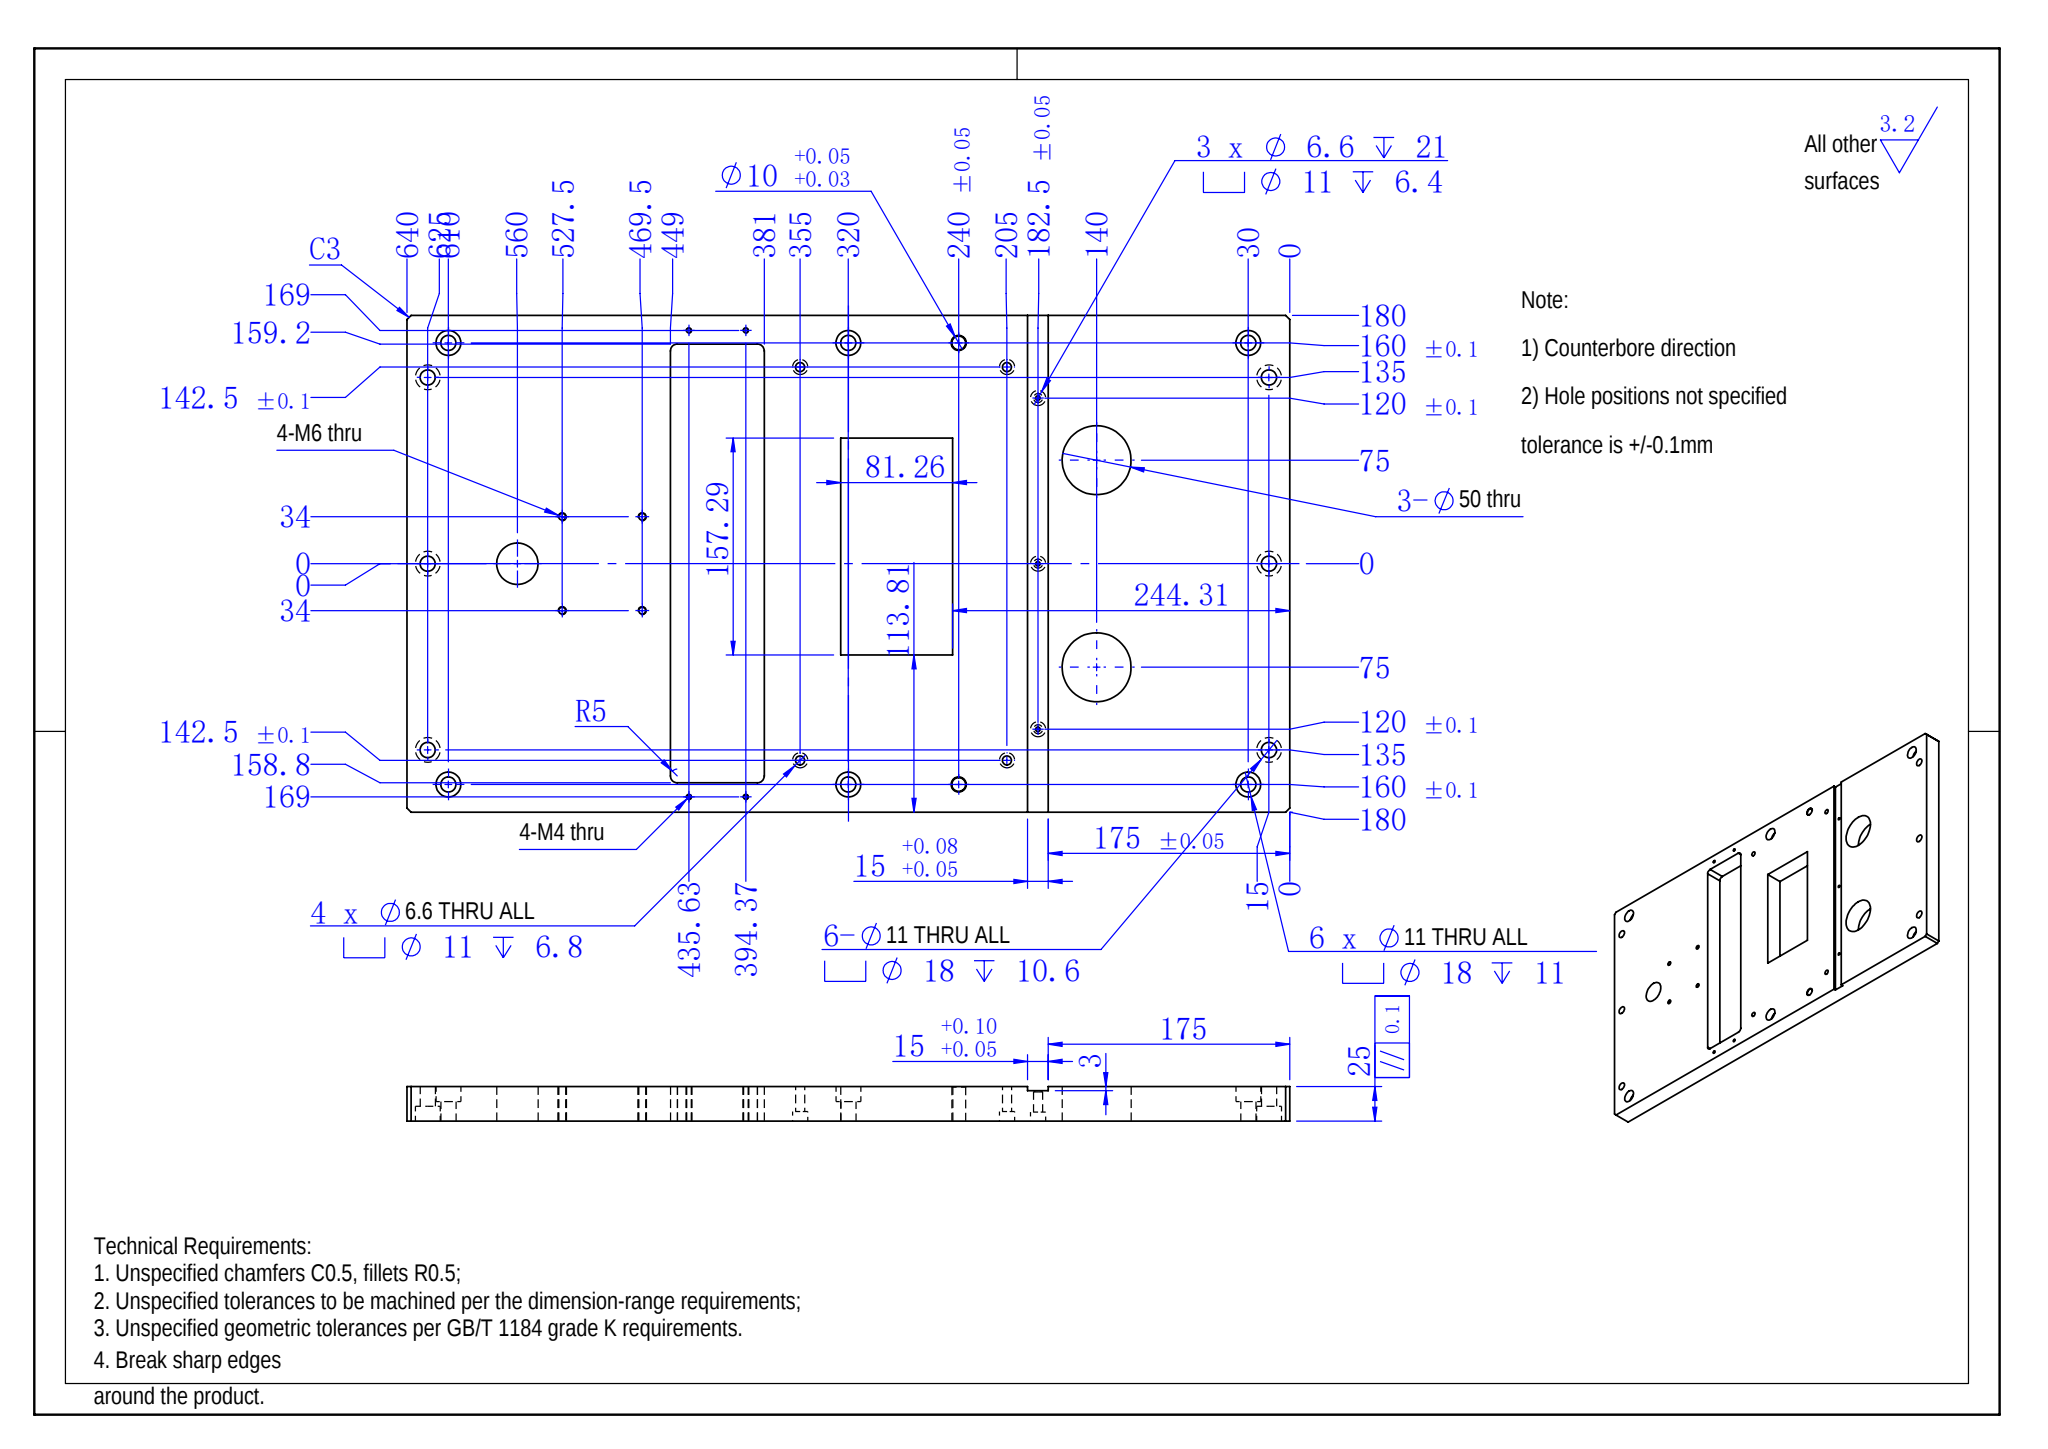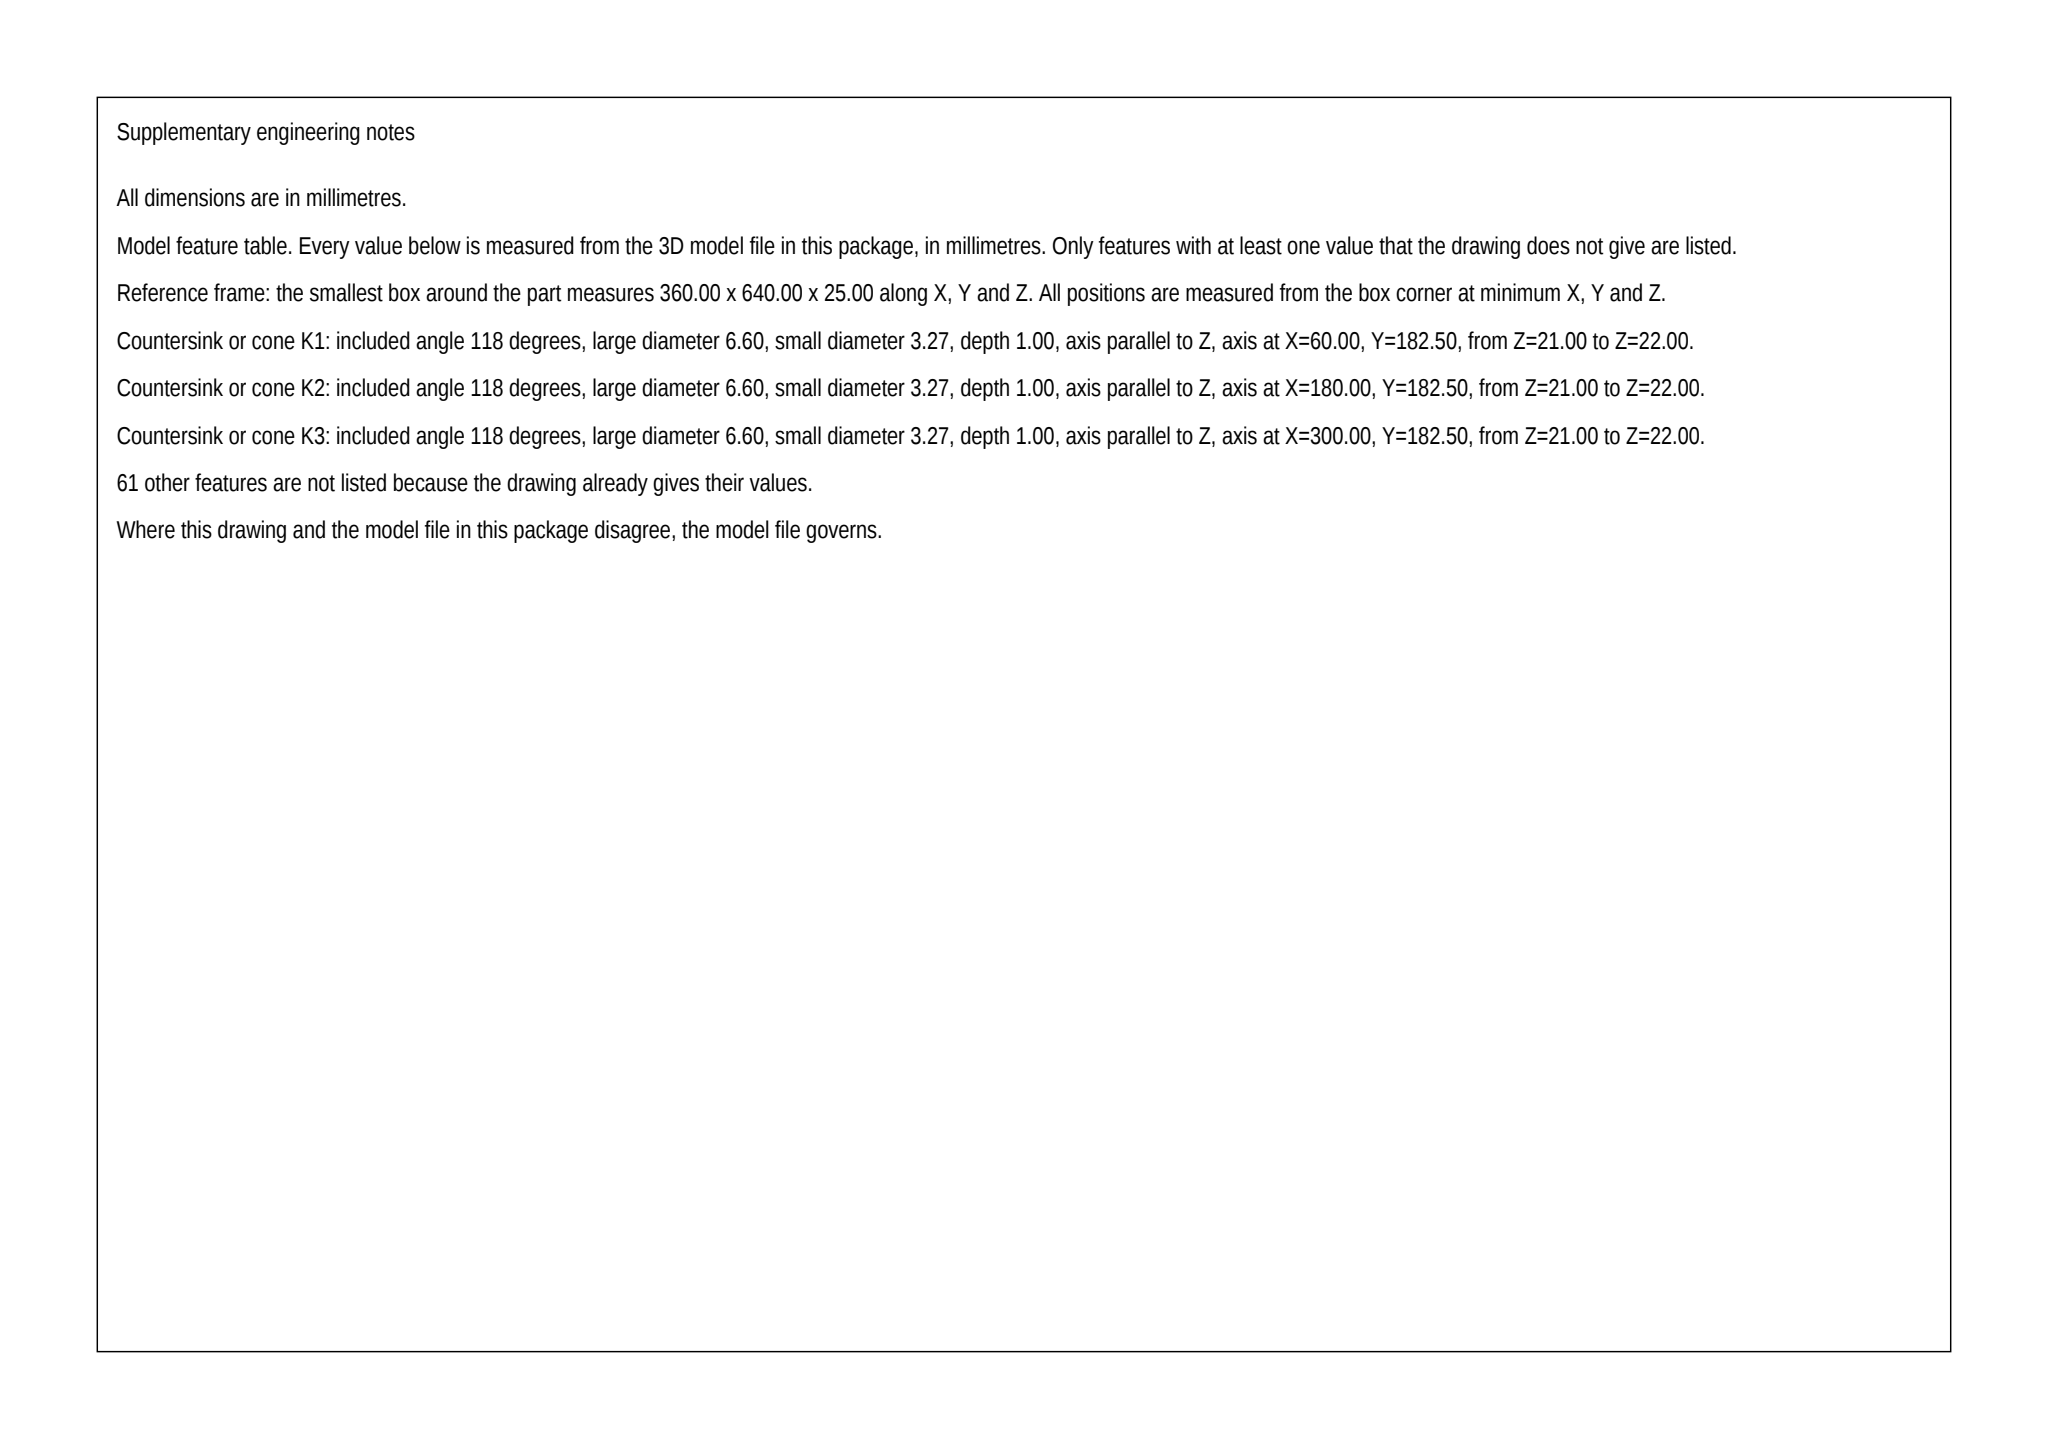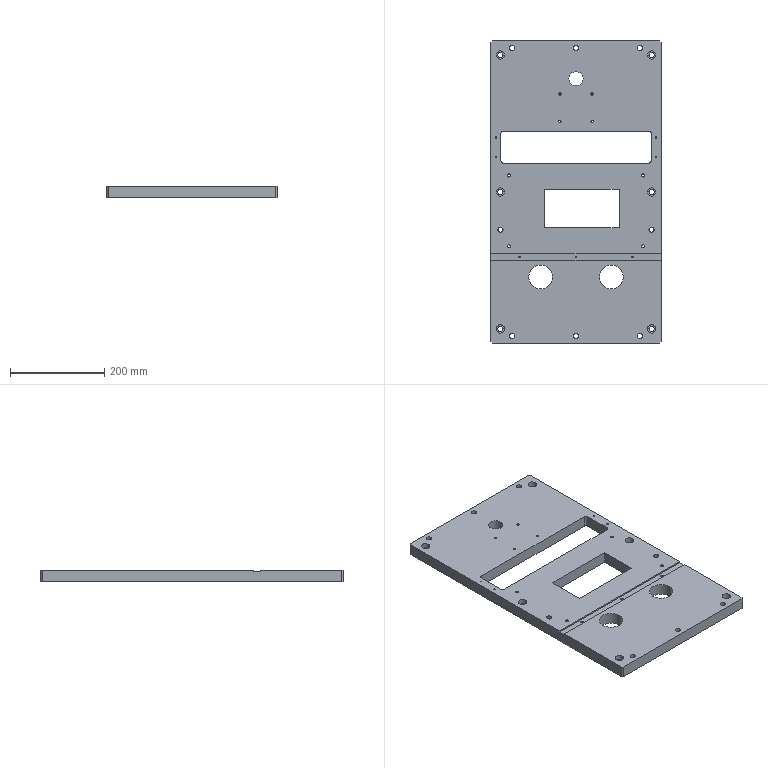Part | SolidWorks | mm | 1 solid | 157 faces | box 360 x 640 x 25 mm | volume 4703508 mm3 | cylinder 106 | plane 41 | cone 10 | commonest cylinder face diameters 11 x38 18 x24 6.6 x14 3.3 x8 5 x8 10 x8 50 x4 30 x2
Drawing notes:
C'BORE DIRECTION: 6X Ø11 THRU WITH C'BORE Ø18 DP 11 (X=20 & 340, Y=30, 320, 610 FROM MIN CORNER) ARE MACHINED FROM THE Z=25 FACE. | from the solid: cylinders [11,z,[20,30],14.0] / [18,z,[20,30],11.0] (also Y320, Y610, X340) with axis_planes z=14.0 count 6 (c'bore floors 25-11)
C'BORE DIRECTION: ALL OTHER C'BORES (Ø18 DP 10.6, Ø11 DP 6.8, Ø11 DP 6.4) ARE MACHINED FROM THE OPPOSITE FACE (Z=0). | from the solid: axis_planes z=10.6 count 6, z=6.8 count 4, z=6.4 count 3 (c'bore floors measured from z=0 face)
2X Ø50 THRU, AT X=105 AND X=255, Y=140 FROM MIN CORNER (NOT 3 HOLES) | from the solid: cylinders: [50.0,"z",[105.0,140.0],25.0] and [50.0,"z",[255.0,140.0],25.0]
1X Ø30 THRU, AT X=180, Y=560 FROM MIN CORNER | from the solid: cylinder: [30.0,"z",[180.0,560.0],25.0]
3X Ø6.6 DP 21, CBORE Ø11 DP 6.4 AT X=60, 180, 300, Y=182.5 FROM MIN CORNER | from the solid: cylinders: [6.6,"z",[60.0/180.0/300.0,182.5],14.6] with [11.0,"z",[60.0/180.0/300.0,182.5],6.4]
6X Ø11 THRU, CBORE Ø18 DP 11 AT X=20 AND 340, Y=30, 320, 610 FROM MIN CORNER | from the solid: cylinders: [11.0,"z",[20.0/340.0,30.0/320.0/610.0],14.0] with [18.0,...,11.0]
6X Ø11 THRU, CBORE Ø18 DP 10.6 AT X=45, 180, 315, Y=15 AND 625 FROM MIN CORNER | from the solid: cylinders: [11.0,"z",[45.0/180.0/315.0,15.0/625.0],14.4] with [18.0,...,10.6]
4X Ø10 THRU AT X=26.2 AND 334.2, Y=386 AND 444 FROM MIN CORNER | from the solid: cylinders: [10.0,"z",[26.2,386.0],25.0], [10.0,"z",[26.2,444.0],25.0], [10.0,"z",[334.2,386.0],25.0], [10.0,"z",[334.2,444.0],25.0]
4X Ø6.6 DP 18.2, CBORE Ø11 DP 6.8 AT X=37.5 AND 322.5, Y=205 AND 355 FROM MIN CORNER | from the solid: cylinders: [6.6,"z",[37.5/322.5,205.0/355.0],18.2] with [11.0,...,6.8]
PLATE OVERALL 640 X 360 X 25 THK; HOLE POSITIONS ABOVE ARE FROM THE MIN-CORNER DATUM | from the solid: bbox_xyz [360.0,640.0,25.0]; origin_note positions from min corner
2X Ø10 (+0.05/+0.03) BLIND HOLE DP 24.5 WITH 90° DRILL POINT, AT X=20 AND X=340, Y=240 FROM MIN CORNER | from the solid: cylinders: Ø10 z-axis at (20,240) and (340,240), from z=0 to 24.5; cones 90° ref dia 10 starting z=24.5
SLOT 318 X 68 WITH R5 CORNERS, THRU 25 THK: X=21.2 TO 339.2, Y=381 TO 449 FROM MIN CORNER | from the solid: axis planes x=21.2 & x=339.2 (y 386-444, z 0-25) and y=381 & y=449 (x 26.2-334.2, z 0-25); 4X Ø10 90° concave corner arcs z 0-25
RECTANGULAR OPENING 157.29 X 81.26 THRU 25 THK: X=113.81 TO 271.10 AND Y=244.31 TO 325.57 FROM MIN CORNER (NOT SYMMETRIC ABOUT PLATE CENTRELINE) | from the solid: axis planes x=113.8 & x=271.1 (y 244.3-325.6, z 0-25) and y=244.3 & y=325.6 (x 113.8-271.1, z 0-25)
RECESS 15 WIDE X 3 DEEP (FLOOR AT Z=22) BETWEEN Y=175 AND Y=190, RUNS FULL PLATE WIDTH X=0 TO 360, OPEN AT BOTH ENDS | from the solid: plane z=22 extent x 0-360, y 175-190; planes y=175 and y=190 extent x 0-360, z 22-25
C3 CHAMFER (3 X 45°) AT ALL 4 PLATE CORNERS, FULL 25 THK (4X) | from the solid: 4 inclined 45° planes size 3x3x25 at bbox_from (0,0,0), (0,637,0), (357,0,0), (357,637,0)
2X Ø50 THRU AT X=105 AND X=255, Y=140 FROM MIN CORNER (2 HOLES, NOT 3) | from the solid: cylinders: Ø50 z-axis holes at (105,140) and (255,140), from z=0 to z=25 (thru 25 thk)
6X Ø11 THRU, C'BORE Ø18 DP 11 FROM Z=25 FACE, AT X=20 AND 340, Y=30, 320 AND 610 FROM MIN CORNER | from the solid: cylinders: Ø11 z=0-14 and Ø18 z=14-25 at (20/340, 30/320/610)
6X Ø11 THRU, C'BORE Ø18 DP 10.6 FROM Z=0 FACE, AT X=45, 180 AND 315, Y=15 AND 625 FROM MIN CORNER | from the solid: cylinders: Ø18 z=0-10.6 and Ø11 z=10.6-25 at (45/180/315, 15/625)
3X Ø6.6 DP 21, C'BORE Ø11 DP 6.4 AT X=60, 180 AND 300, Y=182.5 FROM MIN CORNER (120 APART) | from the solid: cylinders: Ø11 z=0-6.4 and Ø6.6 z=6.4-21 at (60,182.5), (180,182.5), (300,182.5)
build123d program:
from build123d import *

# Parameters (mm, degrees)
SKETCH1_W                                          = 360
SKETCH1_H                                          = 640
EXTRUDE1_DEPTH                                     = 25
CHAMFER1_SIZE                                      = 3
SKETCH15_W                                         = 360
SKETCH15_H                                         = 15
CUT_EXTRUDE10_DEPTH                                = 3
M6_HEX_SOCKET_HEAD_CAP_SCREW_CBORE1_D              = 6.6
M6_HEX_SOCKET_HEAD_CAP_SCREW_CBORE1_DEPTH          = 21
M6_HEX_SOCKET_HEAD_CAP_SCREW_CBORE1_CBORE_D        = 11
M6_HEX_SOCKET_HEAD_CAP_SCREW_CBORE1_CBORE_DEPTH    = 6.4
M6_HEX_SOCKET_HEAD_CAP_SCREW_CBORE1_TIP            = 1.983
HOLE_SIZE_ACCORDING_TO_TYPE_1_OF_HEXAG_D           = 11
HOLE_SIZE_ACCORDING_TO_TYPE_1_OF_HEXAG_CBORE_D     = 18
HOLE_SIZE_ACCORDING_TO_TYPE_1_OF_HEXAG_CBORE_DEPTH = 11
F_10_0_10_DIAMETER_HOLE1_D                         = 10
CHAMFER2_SIZE                                      = 0.5
M10_HEX_SOCKET_HEAD_CAP_SCREW_CBORE1_D             = 11
M10_HEX_SOCKET_HEAD_CAP_SCREW_CBORE1_CBORE_D       = 18
M10_HEX_SOCKET_HEAD_CAP_SCREW_CBORE1_CBORE_DEPTH   = 10.6
MIRROR2_COPY_1_D                                   = 11
MIRROR2_COPY_1_CBORE_D                             = 18
MIRROR2_COPY_1_CBORE_DEPTH                         = 10.6
HOLE_SIZE_ACCORDING_TO_TYPE_2_OF_HEXAG_D           = 6.6
HOLE_SIZE_ACCORDING_TO_TYPE_2_OF_HEXAG_CBORE_D     = 11
HOLE_SIZE_ACCORDING_TO_TYPE_2_OF_HEXAG_CBORE_DEPTH = 6.8
M6_TAPPED_HOLE1_D                                  = 5
M4_TAPPED_HOLE1_D                                  = 3.3
SKETCH36_W                                         = 318
SKETCH36_H                                         = 68
CUT_EXTRUDE11_DEPTH                                = 593.895
FILLET1_R                                          = 5
M10_HEX_SOCKET_HEAD_CAP_SCREW_CBORE2_D             = 11
M10_HEX_SOCKET_HEAD_CAP_SCREW_CBORE2_CBORE_D       = 18
M10_HEX_SOCKET_HEAD_CAP_SCREW_CBORE2_CBORE_DEPTH   = 10.6
SKETCH40_R                                         = 15
CUT_EXTRUDE14_DEPTH                                = 593.895
SKETCH41_R                                         = 25
CUT_EXTRUDE15_DEPTH                                = 593.895
SKETCH43_W                                         = 157.287
SKETCH43_H                                         = 81.265
CUT_EXTRUDE16_DEPTH                                = 253


with BuildPart() as part:
    # Sketch1 → Extrude1 (new body)
    with BuildSketch(Plane.XY):
        with Locations((40, 230)):
            Rectangle(SKETCH1_W, SKETCH1_H)
    extrude(amount=EXTRUDE1_DEPTH)

    # Chamfer1
    chamfer1_edges = [part.edges().sort_by_distance(p)[0] for p in [
        (-140, 550, 12.5),
        (220, 550, 12.5),
        (220, -90, 12.5),
        (-140, -90, 12.5),
    ]]
    chamfer(chamfer1_edges, length=CHAMFER1_SIZE)

    # Sketch15 → Cut-Extrude10 (cut)
    with BuildSketch(Plane.XY.offset(25)):
        with Locations((40, 92.5)):
            Rectangle(SKETCH15_W, SKETCH15_H)
    extrude(amount=-CUT_EXTRUDE10_DEPTH, mode=Mode.SUBTRACT)

    # M6 Hex Socket Head Cap Screw CBORE1
    with Locations(Plane(origin=(0, 0, 0), x_dir=(-1, 0, 0), z_dir=(0, 0, -1))):
        with Locations((80, 92.5), (-40, 92.5), (-160, 92.5)):
            CounterBoreHole(M6_HEX_SOCKET_HEAD_CAP_SCREW_CBORE1_D / 2, M6_HEX_SOCKET_HEAD_CAP_SCREW_CBORE1_CBORE_D / 2, M6_HEX_SOCKET_HEAD_CAP_SCREW_CBORE1_CBORE_DEPTH, depth=M6_HEX_SOCKET_HEAD_CAP_SCREW_CBORE1_DEPTH)
            with Locations((0, 0, -(M6_HEX_SOCKET_HEAD_CAP_SCREW_CBORE1_DEPTH + M6_HEX_SOCKET_HEAD_CAP_SCREW_CBORE1_TIP / 2))):  # 118° drill point
                Cone(0, M6_HEX_SOCKET_HEAD_CAP_SCREW_CBORE1_D / 2, M6_HEX_SOCKET_HEAD_CAP_SCREW_CBORE1_TIP, mode=Mode.SUBTRACT)

    # Hole Size _According to_ Type 1 of Hexag (through all)
    with Locations(Plane.XY.offset(25)):
        with Locations((-120, 520), (-120, 230), (-120, -60), (200, 520), (200, 230), (200, -60)):
            CounterBoreHole(HOLE_SIZE_ACCORDING_TO_TYPE_1_OF_HEXAG_D / 2, HOLE_SIZE_ACCORDING_TO_TYPE_1_OF_HEXAG_CBORE_D / 2, HOLE_SIZE_ACCORDING_TO_TYPE_1_OF_HEXAG_CBORE_DEPTH)

    # 10.0 _10_ Diameter Hole1 (through all)
    with Locations(Plane.XY.offset(25)):
        with Locations((200, 150), (-120, 150)):
            Hole(F_10_0_10_DIAMETER_HOLE1_D / 2)

    # Chamfer2
    chamfer2_edges = [part.edges().sort_by_distance(p)[0] for p in [
        (-115, 150, 25),
        (205, 150, 25),
    ]]
    chamfer(chamfer2_edges, length=CHAMFER2_SIZE)

    # M10 Hex Socket Head Cap Screw CBORE1 (through all)
    with Locations(Plane(origin=(0, 0, 0), x_dir=(-1, 0, 0), z_dir=(0, 0, -1))):
        with Locations((-175, 535)):
            m10_hex_socket_head_cap_screw_cbore1 = CounterBoreHole(M10_HEX_SOCKET_HEAD_CAP_SCREW_CBORE1_D / 2, M10_HEX_SOCKET_HEAD_CAP_SCREW_CBORE1_CBORE_D / 2, M10_HEX_SOCKET_HEAD_CAP_SCREW_CBORE1_CBORE_DEPTH)

    # Mirror1: M10 Hex Socket Head Cap Screw CBORE1 across plane
    add(m10_hex_socket_head_cap_screw_cbore1.mirror(Plane.ZY.offset(-40)), mode=Mode.SUBTRACT)

    # Mirror2: M10 Hex Socket Head Cap Screw CBORE1 across plane
    add(m10_hex_socket_head_cap_screw_cbore1.mirror(Plane.ZX.offset(230)), mode=Mode.SUBTRACT)

    # Mirror2 copy 1 (through all)
    with Locations(Plane(origin=(80, 460, 0), x_dir=(1, 0, 0), z_dir=(0, 0, -1))):
        with Locations((-175, 535)):
            CounterBoreHole(MIRROR2_COPY_1_D / 2, MIRROR2_COPY_1_CBORE_D / 2, MIRROR2_COPY_1_CBORE_DEPTH)

    # Hole Size _According to_ Type 2 of Hexag (through all)
    with Locations(Plane(origin=(0, 0, 0), x_dir=(-1, 0, 0), z_dir=(0, 0, -1))):
        with Locations((-182.5, 265), (-182.5, 115)):
            hole_size_according_to_type_2_of_hexag = CounterBoreHole(HOLE_SIZE_ACCORDING_TO_TYPE_2_OF_HEXAG_D / 2, HOLE_SIZE_ACCORDING_TO_TYPE_2_OF_HEXAG_CBORE_D / 2, HOLE_SIZE_ACCORDING_TO_TYPE_2_OF_HEXAG_CBORE_DEPTH)

    # Mirror3: Hole Size _According to_ Type 2 of Hexag across plane
    add(hole_size_according_to_type_2_of_hexag.mirror(Plane.ZY.offset(-40)), mode=Mode.SUBTRACT)

    # M6 Tapped Hole1 (through all)
    with Locations(Plane.XY.offset(25)):
        with Locations((74, 437.5), (74, 379.5), (6, 437.5), (6, 379.5)):
            Hole(M6_TAPPED_HOLE1_D / 2)

    # M4 Tapped Hole1 (through all)
    with Locations(Plane.XY.offset(25)):
        with Locations((-129, 345.63), (-129, 304.37), (209, 304.37), (209, 345.63)):
            Hole(M4_TAPPED_HOLE1_D / 2)

    # Sketch36 → Cut-Extrude11 (cut, through all)
    with BuildSketch(Plane.XY.offset(25)):
        with Locations((40.2, 325)):
            Rectangle(SKETCH36_W, SKETCH36_H)
    extrude(amount=-CUT_EXTRUDE11_DEPTH, mode=Mode.SUBTRACT)

    # Fillet1
    fillet1_edges = [part.edges().sort_by_distance(p)[0] for p in [
        (-118.8, 291, 12.5),
        (-118.8, 359, 12.5),
        (199.2, 359, 12.5),
        (199.2, 291, 12.5),
    ]]
    fillet(fillet1_edges, radius=FILLET1_R)

    # M10 Hex Socket Head Cap Screw CBORE2 (through all)
    with Locations(Plane(origin=(0, 0, 0), x_dir=(-1, 0, 0), z_dir=(0, 0, -1))):
        with Locations((-40, -75), (-40, 535)):
            CounterBoreHole(M10_HEX_SOCKET_HEAD_CAP_SCREW_CBORE2_D / 2, M10_HEX_SOCKET_HEAD_CAP_SCREW_CBORE2_CBORE_D / 2, M10_HEX_SOCKET_HEAD_CAP_SCREW_CBORE2_CBORE_DEPTH)

    # Sketch40 → Cut-Extrude14 (cut, through all)
    with BuildSketch(Plane.XY.offset(25)):
        with Locations((40, 470)):
            Circle(SKETCH40_R)
    extrude(amount=-CUT_EXTRUDE14_DEPTH, mode=Mode.SUBTRACT)

    # Sketch41 → Cut-Extrude15 (cut, through all)
    with BuildSketch(Plane.XY.offset(25)):
        with Locations((-35, 50)):
            Circle(SKETCH41_R)
        with Locations((115, 50)):
            Circle(SKETCH41_R)
    extrude(amount=-CUT_EXTRUDE15_DEPTH, mode=Mode.SUBTRACT)

    # Sketch43 → Cut-Extrude16 (cut)
    with BuildSketch(Plane.XY.offset(25)):
        with Locations((52.452, 194.938)):
            Rectangle(SKETCH43_W, SKETCH43_H)
    extrude(amount=-CUT_EXTRUDE16_DEPTH, mode=Mode.SUBTRACT)


solid = part.part